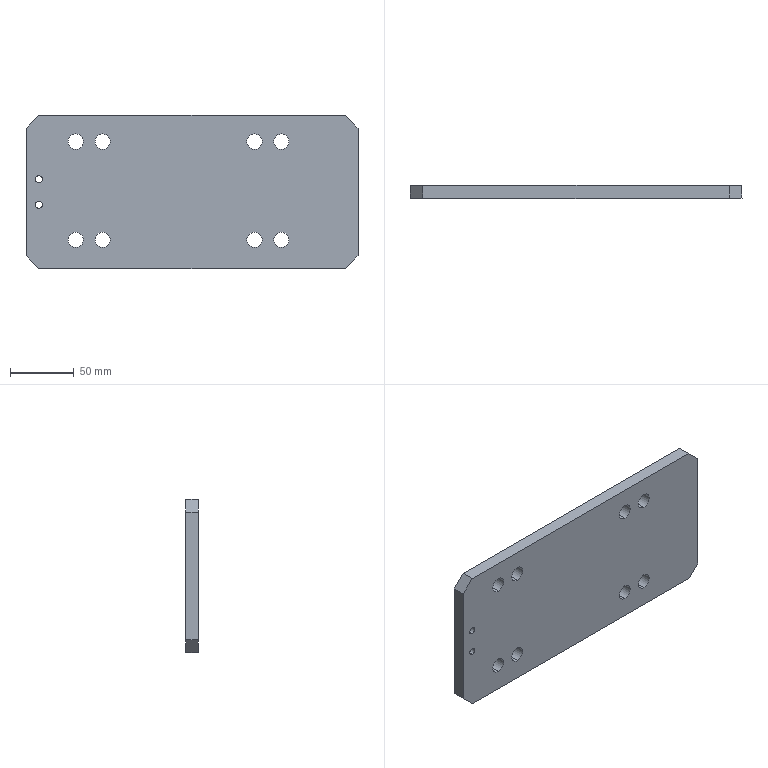Component | SolidWorks | AdsorptionPlate-1 | 1 solid | 30 faces | box 260 x 10.04 x 120 mm | volume 300477 mm3 | cylinder 20 | plane 10 | commonest cylinder face diameters 12 x16 5.5 x4
build123d program:
from build123d import *

# Parameters (mm, degrees)
SKETCH1_W                        = 135
SKETCH1_H                        = 260
BOSS_EXTRUDE1_DEPTH              = 10
M12X1_25_TAPPED_HOLE1_AT_2_COUNT = 2
M12X1_25_TAPPED_HOLE1_AT_2_PITCH = 21
LPATTERN1_COUNT                  = 2
LPATTERN1_PITCH                  = 77
LPATTERN2_COUNT                  = 2
LPATTERN2_PITCH                  = 140
MOVE_FACE1_BY                    = 7.5
MOVE_FACE1_2_BY                  = 7.5
CHAMFER1_SIZE                    = 10
SKETCH4_R                        = 2.75
CUT_EXTRUDE1_DEPTH               = 10


with BuildPart() as part:
    # Sketch1 → Boss-Extrude1 (new body)
    with BuildSketch(Plane.XY):
        Rectangle(SKETCH1_W, SKETCH1_H)
    extrude(amount=BOSS_EXTRUDE1_DEPTH)

    # Sketch2 → M12x1.25 Tapped Hole1 (revolve, cut)
    with BuildSketch(Plane(origin=(37.5, -70, 10), x_dir=(0, -1, 0), z_dir=(1, 0, 0))):
        Polygon((0, 0), (0, 31.355), (6, 27.75), (6, 0), align=None)
    m12x1_25_tapped_hole1 = revolve(axis=Axis((37.5, -70, 16.35), (0, 0, -1)), mode=Mode.SUBTRACT)

    # M12x1.25 Tapped Hole1 at 2: M12x1.25 Tapped Hole1 ×2
    with Locations(*[(0, i * M12X1_25_TAPPED_HOLE1_AT_2_PITCH, 0) for i in range(1, M12X1_25_TAPPED_HOLE1_AT_2_COUNT)]):
        add(m12x1_25_tapped_hole1, mode=Mode.SUBTRACT)

    # LPattern1: M12x1.25 Tapped Hole1 ×2
    with Locations(*[(-i * LPATTERN1_PITCH, 0, 0) for i in range(1, LPATTERN1_COUNT)]):
        add(m12x1_25_tapped_hole1, mode=Mode.SUBTRACT)

    # LPattern1 copy 1 sketch → LPattern1 copy 1 (revolve, cut)
    with BuildSketch(Plane(origin=(-39.5, -49, 10), x_dir=(0, -1, 0), z_dir=(1, 0, 0))):
        Polygon((0, 0), (0, 31.355), (6, 27.75), (6, 0), align=None)
    revolve(axis=Axis((-39.5, -49, 16.35), (0, 0, -1)), mode=Mode.SUBTRACT)

    # LPattern2: M12x1.25 Tapped Hole1 ×2
    with Locations(*[(0, i * LPATTERN2_PITCH, 0) for i in range(1, LPATTERN2_COUNT)]):
        add(m12x1_25_tapped_hole1, mode=Mode.SUBTRACT)

    # LPattern2 copy 1 sketch → LPattern2 copy 1 (revolve, cut)
    with BuildSketch(Plane(origin=(37.5, 91, 10), x_dir=(0, -1, 0), z_dir=(1, 0, 0))):
        Polygon((0, 0), (0, 31.355), (6, 27.75), (6, 0), align=None)
    revolve(axis=Axis((37.5, 91, 16.35), (0, 0, -1)), mode=Mode.SUBTRACT)

    # LPattern2 copy 2 sketch → LPattern2 copy 2 (revolve, cut)
    with BuildSketch(Plane(origin=(-39.5, 70, 10), x_dir=(0, -1, 0), z_dir=(1, 0, 0))):
        Polygon((0, 0), (0, 31.355), (6, 27.75), (6, 0), align=None)
    revolve(axis=Axis((-39.5, 70, 16.35), (0, 0, -1)), mode=Mode.SUBTRACT)

    # LPattern2 copy 3 sketch → LPattern2 copy 3 (revolve, cut)
    with BuildSketch(Plane(origin=(-39.5, 91, 10), x_dir=(0, -1, 0), z_dir=(1, 0, 0))):
        Polygon((0, 0), (0, 31.355), (6, 27.75), (6, 0), align=None)
    revolve(axis=Axis((-39.5, 91, 16.35), (0, 0, -1)), mode=Mode.SUBTRACT)

    # Move Face1: a face moved inward by 7.5
    extrude(part.faces().sort_by_distance((67.5, 0, 5))[0], amount=MOVE_FACE1_BY, dir=(-1, 0, 0), mode=Mode.SUBTRACT)

    # Move Face1 2: a face moved inward by 7.5
    extrude(part.faces().sort_by_distance((-67.5, 0, 5))[0], amount=MOVE_FACE1_2_BY, dir=(1, 0, 0), mode=Mode.SUBTRACT)

    # Chamfer1
    chamfer1_edges = [part.edges().sort_by_distance(p)[0] for p in [
        (-60, 130, 5),
        (60, 130, 5),
        (60, -130, 5),
        (-60, -130, 5),
    ]]
    chamfer(chamfer1_edges, length=CHAMFER1_SIZE)

    # Sketch4 → Cut-Extrude1 (cut)
    with BuildSketch(Plane.XY.offset(10)):
        with Locations((-10, 120)):
            Circle(SKETCH4_R)
        with Locations((10, 120)):
            Circle(SKETCH4_R)
    extrude(amount=-CUT_EXTRUDE1_DEPTH, mode=Mode.SUBTRACT)


solid = part.part

# Placed as in the assembly
solid = solid.moved(Location((1702.164, 3828.72, 1079.241), (-90, -0.008895, 90)))
STEP:
#1=COLOUR_RGB('',0.7922,0.8196,0.9333);
#2=FILL_AREA_STYLE_COLOUR('',#1);
#3=FILL_AREA_STYLE('',(#2));
#4=SURFACE_STYLE_FILL_AREA(#3);
#5=SURFACE_SIDE_STYLE('',(#4));
#6=SURFACE_STYLE_USAGE(.BOTH.,#5);
#7=PRESENTATION_STYLE_ASSIGNMENT((#6));
#8=CARTESIAN_POINT('',(62.29,150.736,41.988));
#9=VERTEX_POINT('',#8);
#10=CARTESIAN_POINT('',(62.29,150.736,42.204));
#11=VERTEX_POINT('',#10);
#12=CARTESIAN_POINT('',(62.29,150.736,42.096));
#13=DIRECTION('',(0.0001552,-1.,0.));
#14=DIRECTION('',(0.,0.,-1.));
#15=AXIS2_PLACEMENT_3D('',#12,#13,#14);
#16=CIRCLE('',#15,0.1083);
#17=EDGE_CURVE('',#9,#11,#16,.T.);
#18=ORIENTED_EDGE('',*,*,#17,.T.);
#19=CARTESIAN_POINT('',(62.29,151.13,42.204));
#20=VERTEX_POINT('',#19);
#21=CARTESIAN_POINT('',(62.29,150.43,42.204));
#22=DIRECTION('',(-0.0001552,1.,-0.));
#23=VECTOR('',#22,39.37);
#24=LINE('',#21,#23);
#25=EDGE_CURVE('',#11,#20,#24,.T.);
#26=ORIENTED_EDGE('',*,*,#25,.T.);
#27=CARTESIAN_POINT('',(62.29,151.13,41.988));
#28=VERTEX_POINT('',#27);
#29=CARTESIAN_POINT('',(62.29,151.13,42.096));
#30=DIRECTION('',(-0.0001552,1.,-0.));
#31=DIRECTION('',(0.,0.,-1.));
#32=AXIS2_PLACEMENT_3D('',#29,#30,#31);
#33=CIRCLE('',#32,0.1083);
#34=EDGE_CURVE('',#20,#28,#33,.T.);
#35=ORIENTED_EDGE('',*,*,#34,.T.);
#36=CARTESIAN_POINT('',(62.29,150.43,41.988));
#37=DIRECTION('',(-0.0001552,1.,-0.));
#38=VECTOR('',#37,39.37);
#39=LINE('',#36,#38);
#40=EDGE_CURVE('',#9,#28,#39,.T.);
#41=ORIENTED_EDGE('',*,*,#40,.F.);
#42=EDGE_LOOP('',(#18,#26,#35,#41));
#43=FACE_OUTER_BOUND('',#42,.T.);
#44=CARTESIAN_POINT('',(62.29,150.43,42.096));
#45=DIRECTION('',(-0.0001552,1.,-0.));
#46=DIRECTION('',(0.,0.,-1.));
#47=AXIS2_PLACEMENT_3D('',#44,#45,#46);
#48=CYLINDRICAL_SURFACE('',#47,0.1083);
#49=ADVANCED_FACE('',(#43),#48,.F.);
#50=CARTESIAN_POINT('',(62.29,150.736,42.775));
#51=VERTEX_POINT('',#50);
#52=CARTESIAN_POINT('',(62.29,150.736,42.992));
#53=VERTEX_POINT('',#52);
#54=CARTESIAN_POINT('',(62.29,150.736,42.884));
#55=DIRECTION('',(0.0001552,-1.,0.));
#56=DIRECTION('',(0.,0.,-1.));
#57=AXIS2_PLACEMENT_3D('',#54,#55,#56);
#58=CIRCLE('',#57,0.1083);
#59=EDGE_CURVE('',#51,#53,#58,.T.);
#60=ORIENTED_EDGE('',*,*,#59,.T.);
#61=CARTESIAN_POINT('',(62.29,151.13,42.992));
#62=VERTEX_POINT('',#61);
#63=CARTESIAN_POINT('',(62.29,150.43,42.992));
#64=DIRECTION('',(-0.0001552,1.,-0.));
#65=VECTOR('',#64,39.37);
#66=LINE('',#63,#65);
#67=EDGE_CURVE('',#53,#62,#66,.T.);
#68=ORIENTED_EDGE('',*,*,#67,.T.);
#69=CARTESIAN_POINT('',(62.29,151.13,42.775));
#70=VERTEX_POINT('',#69);
#71=CARTESIAN_POINT('',(62.29,151.13,42.884));
#72=DIRECTION('',(-0.0001552,1.,-0.));
#73=DIRECTION('',(0.,0.,-1.));
#74=AXIS2_PLACEMENT_3D('',#71,#72,#73);
#75=CIRCLE('',#74,0.1083);
#76=EDGE_CURVE('',#62,#70,#75,.T.);
#77=ORIENTED_EDGE('',*,*,#76,.T.);
#78=CARTESIAN_POINT('',(62.29,150.43,42.775));
#79=DIRECTION('',(-0.0001552,1.,-0.));
#80=VECTOR('',#79,39.37);
#81=LINE('',#78,#80);
#82=EDGE_CURVE('',#51,#70,#81,.T.);
#83=ORIENTED_EDGE('',*,*,#82,.F.);
#84=EDGE_LOOP('',(#60,#68,#77,#83));
#85=FACE_OUTER_BOUND('',#84,.T.);
#86=CARTESIAN_POINT('',(62.29,150.43,42.884));
#87=DIRECTION('',(-0.0001552,1.,-0.));
#88=DIRECTION('',(0.,0.,-1.));
#89=AXIS2_PLACEMENT_3D('',#86,#87,#88);
#90=CYLINDRICAL_SURFACE('',#89,0.1083);
#91=ADVANCED_FACE('',(#85),#90,.F.);
#92=CARTESIAN_POINT('',(64.258,150.737,44.281));
#93=VERTEX_POINT('',#92);
#94=CARTESIAN_POINT('',(64.258,150.737,43.809));
#95=VERTEX_POINT('',#94);
#96=CARTESIAN_POINT('',(64.258,150.737,44.045));
#97=DIRECTION('',(-0.0001552,1.,-0.));
#98=DIRECTION('',(0.,0.,-1.));
#99=AXIS2_PLACEMENT_3D('',#96,#97,#98);
#100=CIRCLE('',#99,0.2362);
#101=EDGE_CURVE('',#93,#95,#100,.T.);
#102=ORIENTED_EDGE('',*,*,#101,.F.);
#103=CARTESIAN_POINT('',(64.258,151.13,44.281));
#104=VERTEX_POINT('',#103);
#105=CARTESIAN_POINT('',(64.258,151.13,44.281));
#106=DIRECTION('',(-0.0001552,1.,-0.));
#107=VECTOR('',#106,39.37);
#108=LINE('',#105,#107);
#109=EDGE_CURVE('',#93,#104,#108,.T.);
#110=ORIENTED_EDGE('',*,*,#109,.T.);
#111=CARTESIAN_POINT('',(64.258,151.13,43.809));
#112=VERTEX_POINT('',#111);
#113=CARTESIAN_POINT('',(64.258,151.13,44.045));
#114=DIRECTION('',(-0.0001552,1.,-0.));
#115=DIRECTION('',(0.,0.,-1.));
#116=AXIS2_PLACEMENT_3D('',#113,#114,#115);
#117=CIRCLE('',#116,0.2362);
#118=EDGE_CURVE('',#104,#112,#117,.T.);
#119=ORIENTED_EDGE('',*,*,#118,.T.);
#120=CARTESIAN_POINT('',(64.258,151.13,43.809));
#121=DIRECTION('',(-0.0001552,1.,-0.));
#122=VECTOR('',#121,39.37);
#123=LINE('',#120,#122);
#124=EDGE_CURVE('',#95,#112,#123,.T.);
#125=ORIENTED_EDGE('',*,*,#124,.F.);
#126=EDGE_LOOP('',(#102,#110,#119,#125));
#127=FACE_OUTER_BOUND('',#126,.T.);
#128=CARTESIAN_POINT('',(64.258,151.13,44.045));
#129=DIRECTION('',(-0.0001552,1.,-0.));
#130=DIRECTION('',(0.,0.,-1.));
#131=AXIS2_PLACEMENT_3D('',#128,#129,#130);
#132=CYLINDRICAL_SURFACE('',#131,0.2362);
#133=ADVANCED_FACE('',(#127),#132,.F.);
#134=CARTESIAN_POINT('',(64.258,150.737,41.25));
#135=VERTEX_POINT('',#134);
#136=CARTESIAN_POINT('',(64.258,150.737,40.777));
#137=VERTEX_POINT('',#136);
#138=CARTESIAN_POINT('',(64.258,150.737,41.013));
#139=DIRECTION('',(-0.0001552,1.,-0.));
#140=DIRECTION('',(0.,0.,-1.));
#141=AXIS2_PLACEMENT_3D('',#138,#139,#140);
#142=CIRCLE('',#141,0.2362);
#143=EDGE_CURVE('',#135,#137,#142,.T.);
#144=ORIENTED_EDGE('',*,*,#143,.F.);
#145=CARTESIAN_POINT('',(64.258,151.13,41.25));
#146=VERTEX_POINT('',#145);
#147=CARTESIAN_POINT('',(64.258,151.13,41.25));
#148=DIRECTION('',(-0.0001552,1.,-0.));
#149=VECTOR('',#148,39.37);
#150=LINE('',#147,#149);
#151=EDGE_CURVE('',#135,#146,#150,.T.);
#152=ORIENTED_EDGE('',*,*,#151,.T.);
#153=CARTESIAN_POINT('',(64.258,151.13,40.777));
#154=VERTEX_POINT('',#153);
#155=CARTESIAN_POINT('',(64.258,151.13,41.013));
#156=DIRECTION('',(-0.0001552,1.,-0.));
#157=DIRECTION('',(0.,0.,-1.));
#158=AXIS2_PLACEMENT_3D('',#155,#156,#157);
#159=CIRCLE('',#158,0.2362);
#160=EDGE_CURVE('',#146,#154,#159,.T.);
#161=ORIENTED_EDGE('',*,*,#160,.T.);
#162=CARTESIAN_POINT('',(64.258,151.13,40.777));
#163=DIRECTION('',(-0.0001552,1.,-0.));
#164=VECTOR('',#163,39.37);
#165=LINE('',#162,#164);
#166=EDGE_CURVE('',#137,#154,#165,.T.);
#167=ORIENTED_EDGE('',*,*,#166,.F.);
#168=EDGE_LOOP('',(#144,#152,#161,#167));
#169=FACE_OUTER_BOUND('',#168,.T.);
#170=CARTESIAN_POINT('',(64.258,151.13,41.013));
#171=DIRECTION('',(-0.0001552,1.,-0.));
#172=DIRECTION('',(0.,0.,-1.));
#173=AXIS2_PLACEMENT_3D('',#170,#171,#172);
#174=CYLINDRICAL_SURFACE('',#173,0.2362);
#175=ADVANCED_FACE('',(#169),#174,.F.);
#176=CARTESIAN_POINT('',(63.432,150.736,41.25));
#177=VERTEX_POINT('',#176);
#178=CARTESIAN_POINT('',(63.432,150.736,40.777));
#179=VERTEX_POINT('',#178);
#180=CARTESIAN_POINT('',(63.432,150.736,41.013));
#181=DIRECTION('',(-0.0001552,1.,-0.));
#182=DIRECTION('',(0.,0.,-1.));
#183=AXIS2_PLACEMENT_3D('',#180,#181,#182);
#184=CIRCLE('',#183,0.2362);
#185=EDGE_CURVE('',#177,#179,#184,.T.);
#186=ORIENTED_EDGE('',*,*,#185,.F.);
#187=CARTESIAN_POINT('',(63.432,151.13,41.25));
#188=VERTEX_POINT('',#187);
#189=CARTESIAN_POINT('',(63.432,151.13,41.25));
#190=DIRECTION('',(-0.0001552,1.,-0.));
#191=VECTOR('',#190,39.37);
#192=LINE('',#189,#191);
#193=EDGE_CURVE('',#177,#188,#192,.T.);
#194=ORIENTED_EDGE('',*,*,#193,.T.);
#195=CARTESIAN_POINT('',(63.432,151.13,40.777));
#196=VERTEX_POINT('',#195);
#197=CARTESIAN_POINT('',(63.432,151.13,41.013));
#198=DIRECTION('',(-0.0001552,1.,-0.));
#199=DIRECTION('',(0.,0.,-1.));
#200=AXIS2_PLACEMENT_3D('',#197,#198,#199);
#201=CIRCLE('',#200,0.2362);
#202=EDGE_CURVE('',#188,#196,#201,.T.);
#203=ORIENTED_EDGE('',*,*,#202,.T.);
#204=CARTESIAN_POINT('',(63.432,151.13,40.777));
#205=DIRECTION('',(-0.0001552,1.,-0.));
#206=VECTOR('',#205,39.37);
#207=LINE('',#204,#206);
#208=EDGE_CURVE('',#179,#196,#207,.T.);
#209=ORIENTED_EDGE('',*,*,#208,.F.);
#210=EDGE_LOOP('',(#186,#194,#203,#209));
#211=FACE_OUTER_BOUND('',#210,.T.);
#212=CARTESIAN_POINT('',(63.432,151.13,41.013));
#213=DIRECTION('',(-0.0001552,1.,-0.));
#214=DIRECTION('',(0.,0.,-1.));
#215=AXIS2_PLACEMENT_3D('',#212,#213,#214);
#216=CYLINDRICAL_SURFACE('',#215,0.2362);
#217=ADVANCED_FACE('',(#211),#216,.F.);
#218=CARTESIAN_POINT('',(63.432,150.736,44.281));
#219=VERTEX_POINT('',#218);
#220=CARTESIAN_POINT('',(63.432,150.736,43.809));
#221=VERTEX_POINT('',#220);
#222=CARTESIAN_POINT('',(63.432,150.736,44.045));
#223=DIRECTION('',(-0.0001552,1.,-0.));
#224=DIRECTION('',(0.,0.,-1.));
#225=AXIS2_PLACEMENT_3D('',#222,#223,#224);
#226=CIRCLE('',#225,0.2362);
#227=EDGE_CURVE('',#219,#221,#226,.T.);
#228=ORIENTED_EDGE('',*,*,#227,.F.);
#229=CARTESIAN_POINT('',(63.432,151.13,44.281));
#230=VERTEX_POINT('',#229);
#231=CARTESIAN_POINT('',(63.432,151.13,44.281));
#232=DIRECTION('',(-0.0001552,1.,-0.));
#233=VECTOR('',#232,39.37);
#234=LINE('',#231,#233);
#235=EDGE_CURVE('',#219,#230,#234,.T.);
#236=ORIENTED_EDGE('',*,*,#235,.T.);
#237=CARTESIAN_POINT('',(63.432,151.13,43.809));
#238=VERTEX_POINT('',#237);
#239=CARTESIAN_POINT('',(63.432,151.13,44.045));
#240=DIRECTION('',(-0.0001552,1.,-0.));
#241=DIRECTION('',(0.,0.,-1.));
#242=AXIS2_PLACEMENT_3D('',#239,#240,#241);
#243=CIRCLE('',#242,0.2362);
#244=EDGE_CURVE('',#230,#238,#243,.T.);
#245=ORIENTED_EDGE('',*,*,#244,.T.);
#246=CARTESIAN_POINT('',(63.432,151.13,43.809));
#247=DIRECTION('',(-0.0001552,1.,-0.));
#248=VECTOR('',#247,39.37);
#249=LINE('',#246,#248);
#250=EDGE_CURVE('',#221,#238,#249,.T.);
#251=ORIENTED_EDGE('',*,*,#250,.F.);
#252=EDGE_LOOP('',(#228,#236,#245,#251));
#253=FACE_OUTER_BOUND('',#252,.T.);
#254=CARTESIAN_POINT('',(63.432,151.13,44.045));
#255=DIRECTION('',(-0.0001552,1.,-0.));
#256=DIRECTION('',(0.,0.,-1.));
#257=AXIS2_PLACEMENT_3D('',#254,#255,#256);
#258=CYLINDRICAL_SURFACE('',#257,0.2362);
#259=ADVANCED_FACE('',(#253),#258,.F.);
#260=CARTESIAN_POINT('',(68.943,150.737,44.281));
#261=VERTEX_POINT('',#260);
#262=CARTESIAN_POINT('',(68.943,150.737,43.809));
#263=VERTEX_POINT('',#262);
#264=CARTESIAN_POINT('',(68.943,150.737,44.045));
#265=DIRECTION('',(-0.0001552,1.,-0.));
#266=DIRECTION('',(0.,0.,-1.));
#267=AXIS2_PLACEMENT_3D('',#264,#265,#266);
#268=CIRCLE('',#267,0.2362);
#269=EDGE_CURVE('',#261,#263,#268,.T.);
#270=ORIENTED_EDGE('',*,*,#269,.F.);
#271=CARTESIAN_POINT('',(68.943,151.131,44.281));
#272=VERTEX_POINT('',#271);
#273=CARTESIAN_POINT('',(68.943,151.131,44.281));
#274=DIRECTION('',(-0.0001552,1.,-0.));
#275=VECTOR('',#274,39.37);
#276=LINE('',#273,#275);
#277=EDGE_CURVE('',#261,#272,#276,.T.);
#278=ORIENTED_EDGE('',*,*,#277,.T.);
#279=CARTESIAN_POINT('',(68.943,151.131,43.809));
#280=VERTEX_POINT('',#279);
#281=CARTESIAN_POINT('',(68.943,151.131,44.045));
#282=DIRECTION('',(-0.0001552,1.,-0.));
#283=DIRECTION('',(0.,0.,-1.));
#284=AXIS2_PLACEMENT_3D('',#281,#282,#283);
#285=CIRCLE('',#284,0.2362);
#286=EDGE_CURVE('',#272,#280,#285,.T.);
#287=ORIENTED_EDGE('',*,*,#286,.T.);
#288=CARTESIAN_POINT('',(68.943,151.131,43.809));
#289=DIRECTION('',(-0.0001552,1.,-0.));
#290=VECTOR('',#289,39.37);
#291=LINE('',#288,#290);
#292=EDGE_CURVE('',#263,#280,#291,.T.);
#293=ORIENTED_EDGE('',*,*,#292,.F.);
#294=EDGE_LOOP('',(#270,#278,#287,#293));
#295=FACE_OUTER_BOUND('',#294,.T.);
#296=CARTESIAN_POINT('',(68.943,151.131,44.045));
#297=DIRECTION('',(-0.0001552,1.,-0.));
#298=DIRECTION('',(0.,0.,-1.));
#299=AXIS2_PLACEMENT_3D('',#296,#297,#298);
#300=CYLINDRICAL_SURFACE('',#299,0.2362);
#301=ADVANCED_FACE('',(#295),#300,.F.);
#302=CARTESIAN_POINT('',(69.77,150.737,44.281));
#303=VERTEX_POINT('',#302);
#304=CARTESIAN_POINT('',(69.77,150.737,43.809));
#305=VERTEX_POINT('',#304);
#306=CARTESIAN_POINT('',(69.77,150.737,44.045));
#307=DIRECTION('',(-0.0001552,1.,-0.));
#308=DIRECTION('',(0.,0.,-1.));
#309=AXIS2_PLACEMENT_3D('',#306,#307,#308);
#310=CIRCLE('',#309,0.2362);
#311=EDGE_CURVE('',#303,#305,#310,.T.);
#312=ORIENTED_EDGE('',*,*,#311,.F.);
#313=CARTESIAN_POINT('',(69.77,151.131,44.281));
#314=VERTEX_POINT('',#313);
#315=CARTESIAN_POINT('',(69.77,151.131,44.281));
#316=DIRECTION('',(-0.0001552,1.,-0.));
#317=VECTOR('',#316,39.37);
#318=LINE('',#315,#317);
#319=EDGE_CURVE('',#303,#314,#318,.T.);
#320=ORIENTED_EDGE('',*,*,#319,.T.);
#321=CARTESIAN_POINT('',(69.77,151.131,43.809));
#322=VERTEX_POINT('',#321);
#323=CARTESIAN_POINT('',(69.77,151.131,44.045));
#324=DIRECTION('',(-0.0001552,1.,-0.));
#325=DIRECTION('',(0.,0.,-1.));
#326=AXIS2_PLACEMENT_3D('',#323,#324,#325);
#327=CIRCLE('',#326,0.2362);
#328=EDGE_CURVE('',#314,#322,#327,.T.);
#329=ORIENTED_EDGE('',*,*,#328,.T.);
#330=CARTESIAN_POINT('',(69.77,151.131,43.809));
#331=DIRECTION('',(-0.0001552,1.,-0.));
#332=VECTOR('',#331,39.37);
#333=LINE('',#330,#332);
#334=EDGE_CURVE('',#305,#322,#333,.T.);
#335=ORIENTED_EDGE('',*,*,#334,.F.);
#336=EDGE_LOOP('',(#312,#320,#329,#335));
#337=FACE_OUTER_BOUND('',#336,.T.);
#338=CARTESIAN_POINT('',(69.77,151.131,44.045));
#339=DIRECTION('',(-0.0001552,1.,-0.));
#340=DIRECTION('',(0.,0.,-1.));
#341=AXIS2_PLACEMENT_3D('',#338,#339,#340);
#342=CYLINDRICAL_SURFACE('',#341,0.2362);
#343=ADVANCED_FACE('',(#337),#342,.F.);
#344=CARTESIAN_POINT('',(69.77,150.737,41.25));
#345=VERTEX_POINT('',#344);
#346=CARTESIAN_POINT('',(69.77,150.737,40.777));
#347=VERTEX_POINT('',#346);
#348=CARTESIAN_POINT('',(69.77,150.737,41.013));
#349=DIRECTION('',(-0.0001552,1.,-0.));
#350=DIRECTION('',(0.,0.,-1.));
#351=AXIS2_PLACEMENT_3D('',#348,#349,#350);
#352=CIRCLE('',#351,0.2362);
#353=EDGE_CURVE('',#345,#347,#352,.T.);
#354=ORIENTED_EDGE('',*,*,#353,.F.);
#355=CARTESIAN_POINT('',(69.77,151.131,41.25));
#356=VERTEX_POINT('',#355);
#357=CARTESIAN_POINT('',(69.77,151.131,41.25));
#358=DIRECTION('',(-0.0001552,1.,-0.));
#359=VECTOR('',#358,39.37);
#360=LINE('',#357,#359);
#361=EDGE_CURVE('',#345,#356,#360,.T.);
#362=ORIENTED_EDGE('',*,*,#361,.T.);
#363=CARTESIAN_POINT('',(69.77,151.131,40.777));
#364=VERTEX_POINT('',#363);
#365=CARTESIAN_POINT('',(69.77,151.131,41.013));
#366=DIRECTION('',(-0.0001552,1.,-0.));
#367=DIRECTION('',(0.,0.,-1.));
#368=AXIS2_PLACEMENT_3D('',#365,#366,#367);
#369=CIRCLE('',#368,0.2362);
#370=EDGE_CURVE('',#356,#364,#369,.T.);
#371=ORIENTED_EDGE('',*,*,#370,.T.);
#372=CARTESIAN_POINT('',(69.77,151.131,40.777));
#373=DIRECTION('',(-0.0001552,1.,-0.));
#374=VECTOR('',#373,39.37);
#375=LINE('',#372,#374);
#376=EDGE_CURVE('',#347,#364,#375,.T.);
#377=ORIENTED_EDGE('',*,*,#376,.F.);
#378=EDGE_LOOP('',(#354,#362,#371,#377));
#379=FACE_OUTER_BOUND('',#378,.T.);
#380=CARTESIAN_POINT('',(69.77,151.131,41.013));
#381=DIRECTION('',(-0.0001552,1.,-0.));
#382=DIRECTION('',(0.,0.,-1.));
#383=AXIS2_PLACEMENT_3D('',#380,#381,#382);
#384=CYLINDRICAL_SURFACE('',#383,0.2362);
#385=ADVANCED_FACE('',(#379),#384,.F.);
#386=CARTESIAN_POINT('',(68.943,150.737,41.25));
#387=VERTEX_POINT('',#386);
#388=CARTESIAN_POINT('',(68.943,150.737,40.777));
#389=VERTEX_POINT('',#388);
#390=CARTESIAN_POINT('',(68.943,150.737,41.013));
#391=DIRECTION('',(-0.0001552,1.,-0.));
#392=DIRECTION('',(0.,0.,-1.));
#393=AXIS2_PLACEMENT_3D('',#390,#391,#392);
#394=CIRCLE('',#393,0.2362);
#395=EDGE_CURVE('',#387,#389,#394,.T.);
#396=ORIENTED_EDGE('',*,*,#395,.F.);
#397=CARTESIAN_POINT('',(68.943,151.131,41.25));
#398=VERTEX_POINT('',#397);
#399=CARTESIAN_POINT('',(68.943,151.131,41.25));
#400=DIRECTION('',(-0.0001552,1.,-0.));
#401=VECTOR('',#400,39.37);
#402=LINE('',#399,#401);
#403=EDGE_CURVE('',#387,#398,#402,.T.);
#404=ORIENTED_EDGE('',*,*,#403,.T.);
#405=CARTESIAN_POINT('',(68.943,151.131,40.777));
#406=VERTEX_POINT('',#405);
#407=CARTESIAN_POINT('',(68.943,151.131,41.013));
#408=DIRECTION('',(-0.0001552,1.,-0.));
#409=DIRECTION('',(0.,0.,-1.));
#410=AXIS2_PLACEMENT_3D('',#407,#408,#409);
#411=CIRCLE('',#410,0.2362);
#412=EDGE_CURVE('',#398,#406,#411,.T.);
#413=ORIENTED_EDGE('',*,*,#412,.T.);
#414=CARTESIAN_POINT('',(68.943,151.131,40.777));
#415=DIRECTION('',(-0.0001552,1.,-0.));
#416=VECTOR('',#415,39.37);
#417=LINE('',#414,#416);
#418=EDGE_CURVE('',#389,#406,#417,.T.);
#419=ORIENTED_EDGE('',*,*,#418,.F.);
#420=EDGE_LOOP('',(#396,#404,#413,#419));
#421=FACE_OUTER_BOUND('',#420,.T.);
#422=CARTESIAN_POINT('',(68.943,151.131,41.013));
#423=DIRECTION('',(-0.0001552,1.,-0.));
#424=DIRECTION('',(0.,0.,-1.));
#425=AXIS2_PLACEMENT_3D('',#422,#423,#424);
#426=CYLINDRICAL_SURFACE('',#425,0.2362);
#427=ADVANCED_FACE('',(#421),#426,.F.);
#428=CARTESIAN_POINT('',(62.29,151.13,44.852));
#429=VERTEX_POINT('',#428);
#430=CARTESIAN_POINT('',(71.739,151.131,44.852));
#431=VERTEX_POINT('',#430);
#432=CARTESIAN_POINT('',(72.132,151.132,44.852));
#433=DIRECTION('',(1.,0.0001552,0.));
#434=VECTOR('',#433,39.37);
#435=LINE('',#432,#434);
#436=EDGE_CURVE('',#429,#431,#435,.T.);
#437=ORIENTED_EDGE('',*,*,#436,.F.);
#438=CARTESIAN_POINT('',(62.29,150.736,44.852));
#439=VERTEX_POINT('',#438);
#440=CARTESIAN_POINT('',(62.29,151.13,44.852));
#441=DIRECTION('',(0.0001552,-1.,0.));
#442=VECTOR('',#441,39.37);
#443=LINE('',#440,#442);
#444=EDGE_CURVE('',#429,#439,#443,.T.);
#445=ORIENTED_EDGE('',*,*,#444,.T.);
#446=CARTESIAN_POINT('',(71.739,150.738,44.852));
#447=VERTEX_POINT('',#446);
#448=CARTESIAN_POINT('',(72.132,150.738,44.852));
#449=DIRECTION('',(1.,0.0001552,0.));
#450=VECTOR('',#449,39.37);
#451=LINE('',#448,#450);
#452=EDGE_CURVE('',#439,#447,#451,.T.);
#453=ORIENTED_EDGE('',*,*,#452,.T.);
#454=CARTESIAN_POINT('',(71.739,151.131,44.852));
#455=DIRECTION('',(-0.0001552,1.,-0.));
#456=VECTOR('',#455,39.37);
#457=LINE('',#454,#456);
#458=EDGE_CURVE('',#447,#431,#457,.T.);
#459=ORIENTED_EDGE('',*,*,#458,.T.);
#460=EDGE_LOOP('',(#437,#445,#453,#459));
#461=FACE_OUTER_BOUND('',#460,.T.);
#462=CARTESIAN_POINT('',(72.132,151.132,44.852));
#463=DIRECTION('',(0.,-0.,-1.));
#464=DIRECTION('',(0.0001552,-1.,0.));
#465=AXIS2_PLACEMENT_3D('',#462,#463,#464);
#466=PLANE('',#465);
#467=ADVANCED_FACE('',(#461),#466,.F.);
#468=CARTESIAN_POINT('',(72.132,150.738,44.458));
#469=VERTEX_POINT('',#468);
#470=CARTESIAN_POINT('',(72.132,150.738,40.521));
#471=VERTEX_POINT('',#470);
#472=CARTESIAN_POINT('',(72.132,150.738,39.832));
#473=DIRECTION('',(0.,-0.,-1.));
#474=VECTOR('',#473,39.37);
#475=LINE('',#472,#474);
#476=EDGE_CURVE('',#469,#471,#475,.T.);
#477=ORIENTED_EDGE('',*,*,#476,.T.);
#478=CARTESIAN_POINT('',(72.132,151.132,40.521));
#479=VERTEX_POINT('',#478);
#480=CARTESIAN_POINT('',(72.132,151.132,40.521));
#481=DIRECTION('',(-0.0001552,1.,-0.));
#482=VECTOR('',#481,39.37);
#483=LINE('',#480,#482);
#484=EDGE_CURVE('',#471,#479,#483,.T.);
#485=ORIENTED_EDGE('',*,*,#484,.T.);
#486=CARTESIAN_POINT('',(72.132,151.132,44.458));
#487=VERTEX_POINT('',#486);
#488=CARTESIAN_POINT('',(72.132,151.132,39.832));
#489=DIRECTION('',(0.,-0.,-1.));
#490=VECTOR('',#489,39.37);
#491=LINE('',#488,#490);
#492=EDGE_CURVE('',#487,#479,#491,.T.);
#493=ORIENTED_EDGE('',*,*,#492,.F.);
#494=CARTESIAN_POINT('',(72.132,151.132,44.458));
#495=DIRECTION('',(0.0001552,-1.,0.));
#496=VECTOR('',#495,39.37);
#497=LINE('',#494,#496);
#498=EDGE_CURVE('',#487,#469,#497,.T.);
#499=ORIENTED_EDGE('',*,*,#498,.T.);
#500=EDGE_LOOP('',(#477,#485,#493,#499));
#501=FACE_OUTER_BOUND('',#500,.T.);
#502=CARTESIAN_POINT('',(72.132,151.132,39.832));
#503=DIRECTION('',(-1.,-0.0001552,-0.));
#504=DIRECTION('',(-0.0001552,1.,-0.));
#505=AXIS2_PLACEMENT_3D('',#502,#503,#504);
#506=PLANE('',#505);
#507=ADVANCED_FACE('',(#501),#506,.F.);
#508=CARTESIAN_POINT('',(71.739,150.738,40.128));
#509=VERTEX_POINT('',#508);
#510=CARTESIAN_POINT('',(62.29,150.736,40.128));
#511=VERTEX_POINT('',#510);
#512=CARTESIAN_POINT('',(72.132,150.738,40.128));
#513=DIRECTION('',(-1.,-0.0001552,-0.));
#514=VECTOR('',#513,39.37);
#515=LINE('',#512,#514);
#516=EDGE_CURVE('',#509,#511,#515,.T.);
#517=ORIENTED_EDGE('',*,*,#516,.T.);
#518=CARTESIAN_POINT('',(62.29,151.13,40.128));
#519=VERTEX_POINT('',#518);
#520=CARTESIAN_POINT('',(62.29,151.13,40.128));
#521=DIRECTION('',(-0.0001552,1.,-0.));
#522=VECTOR('',#521,39.37);
#523=LINE('',#520,#522);
#524=EDGE_CURVE('',#511,#519,#523,.T.);
#525=ORIENTED_EDGE('',*,*,#524,.T.);
#526=CARTESIAN_POINT('',(71.739,151.131,40.128));
#527=VERTEX_POINT('',#526);
#528=CARTESIAN_POINT('',(72.132,151.132,40.128));
#529=DIRECTION('',(-1.,-0.0001552,-0.));
#530=VECTOR('',#529,39.37);
#531=LINE('',#528,#530);
#532=EDGE_CURVE('',#527,#519,#531,.T.);
#533=ORIENTED_EDGE('',*,*,#532,.F.);
#534=CARTESIAN_POINT('',(71.739,151.131,40.128));
#535=DIRECTION('',(0.0001552,-1.,0.));
#536=VECTOR('',#535,39.37);
#537=LINE('',#534,#536);
#538=EDGE_CURVE('',#527,#509,#537,.T.);
#539=ORIENTED_EDGE('',*,*,#538,.T.);
#540=EDGE_LOOP('',(#517,#525,#533,#539));
#541=FACE_OUTER_BOUND('',#540,.T.);
#542=CARTESIAN_POINT('',(72.132,151.132,40.128));
#543=DIRECTION('',(-0.,0.,1.));
#544=DIRECTION('',(-0.0001552,1.,-0.));
#545=AXIS2_PLACEMENT_3D('',#542,#543,#544);
#546=PLANE('',#545);
#547=ADVANCED_FACE('',(#541),#546,.F.);
#548=CARTESIAN_POINT('',(61.896,150.736,40.521));
#549=VERTEX_POINT('',#548);
#550=CARTESIAN_POINT('',(61.896,150.736,44.458));
#551=VERTEX_POINT('',#550);
#552=CARTESIAN_POINT('',(61.896,150.736,39.832));
#553=DIRECTION('',(0.,0.,1.));
#554=VECTOR('',#553,39.37);
#555=LINE('',#552,#554);
#556=EDGE_CURVE('',#549,#551,#555,.T.);
#557=ORIENTED_EDGE('',*,*,#556,.T.);
#558=CARTESIAN_POINT('',(61.896,151.13,44.458));
#559=VERTEX_POINT('',#558);
#560=CARTESIAN_POINT('',(61.896,151.13,44.458));
#561=DIRECTION('',(-0.0001552,1.,-0.));
#562=VECTOR('',#561,39.37);
#563=LINE('',#560,#562);
#564=EDGE_CURVE('',#551,#559,#563,.T.);
#565=ORIENTED_EDGE('',*,*,#564,.T.);
#566=CARTESIAN_POINT('',(61.896,151.13,40.521));
#567=VERTEX_POINT('',#566);
#568=CARTESIAN_POINT('',(61.896,151.13,39.832));
#569=DIRECTION('',(0.,0.,1.));
#570=VECTOR('',#569,39.37);
#571=LINE('',#568,#570);
#572=EDGE_CURVE('',#567,#559,#571,.T.);
#573=ORIENTED_EDGE('',*,*,#572,.F.);
#574=CARTESIAN_POINT('',(61.896,151.13,40.521));
#575=DIRECTION('',(0.0001552,-1.,0.));
#576=VECTOR('',#575,39.37);
#577=LINE('',#574,#576);
#578=EDGE_CURVE('',#567,#549,#577,.T.);
#579=ORIENTED_EDGE('',*,*,#578,.T.);
#580=EDGE_LOOP('',(#557,#565,#573,#579));
#581=FACE_OUTER_BOUND('',#580,.T.);
#582=CARTESIAN_POINT('',(61.896,151.13,39.832));
#583=DIRECTION('',(1.,0.0001552,-0.));
#584=DIRECTION('',(-0.,-0.,-1.));
#585=AXIS2_PLACEMENT_3D('',#582,#583,#584);
#586=PLANE('',#585);
#587=ADVANCED_FACE('',(#581),#586,.F.);
#588=CARTESIAN_POINT('',(62.29,151.13,42.096));
#589=DIRECTION('',(-0.0001552,1.,-0.));
#590=DIRECTION('',(0.,0.,-1.));
#591=AXIS2_PLACEMENT_3D('',#588,#589,#590);
#592=CIRCLE('',#591,0.1083);
#593=EDGE_CURVE('',#28,#20,#592,.T.);
#594=ORIENTED_EDGE('',*,*,#593,.F.);
#595=ORIENTED_EDGE('',*,*,#34,.F.);
#596=EDGE_LOOP('',(#594,#595));
#597=FACE_BOUND('',#596,.T.);
#598=CARTESIAN_POINT('',(62.29,151.13,42.884));
#599=DIRECTION('',(-0.0001552,1.,-0.));
#600=DIRECTION('',(0.,0.,-1.));
#601=AXIS2_PLACEMENT_3D('',#598,#599,#600);
#602=CIRCLE('',#601,0.1083);
#603=EDGE_CURVE('',#70,#62,#602,.T.);
#604=ORIENTED_EDGE('',*,*,#603,.F.);
#605=ORIENTED_EDGE('',*,*,#76,.F.);
#606=EDGE_LOOP('',(#604,#605));
#607=FACE_BOUND('',#606,.T.);
#608=CARTESIAN_POINT('',(64.258,151.13,44.045));
#609=DIRECTION('',(-0.0001552,1.,-0.));
#610=DIRECTION('',(0.,0.,-1.));
#611=AXIS2_PLACEMENT_3D('',#608,#609,#610);
#612=CIRCLE('',#611,0.2362);
#613=EDGE_CURVE('',#112,#104,#612,.T.);
#614=ORIENTED_EDGE('',*,*,#613,.F.);
#615=ORIENTED_EDGE('',*,*,#118,.F.);
#616=EDGE_LOOP('',(#614,#615));
#617=FACE_BOUND('',#616,.T.);
#618=CARTESIAN_POINT('',(64.258,151.13,41.013));
#619=DIRECTION('',(-0.0001552,1.,-0.));
#620=DIRECTION('',(0.,0.,-1.));
#621=AXIS2_PLACEMENT_3D('',#618,#619,#620);
#622=CIRCLE('',#621,0.2362);
#623=EDGE_CURVE('',#154,#146,#622,.T.);
#624=ORIENTED_EDGE('',*,*,#623,.F.);
#625=ORIENTED_EDGE('',*,*,#160,.F.);
#626=EDGE_LOOP('',(#624,#625));
#627=FACE_BOUND('',#626,.T.);
#628=CARTESIAN_POINT('',(63.432,151.13,41.013));
#629=DIRECTION('',(-0.0001552,1.,-0.));
#630=DIRECTION('',(0.,0.,-1.));
#631=AXIS2_PLACEMENT_3D('',#628,#629,#630);
#632=CIRCLE('',#631,0.2362);
#633=EDGE_CURVE('',#196,#188,#632,.T.);
#634=ORIENTED_EDGE('',*,*,#633,.F.);
#635=ORIENTED_EDGE('',*,*,#202,.F.);
#636=EDGE_LOOP('',(#634,#635));
#637=FACE_BOUND('',#636,.T.);
#638=CARTESIAN_POINT('',(63.432,151.13,44.045));
#639=DIRECTION('',(-0.0001552,1.,-0.));
#640=DIRECTION('',(0.,0.,-1.));
#641=AXIS2_PLACEMENT_3D('',#638,#639,#640);
#642=CIRCLE('',#641,0.2362);
#643=EDGE_CURVE('',#238,#230,#642,.T.);
#644=ORIENTED_EDGE('',*,*,#643,.F.);
#645=ORIENTED_EDGE('',*,*,#244,.F.);
#646=EDGE_LOOP('',(#644,#645));
#647=FACE_BOUND('',#646,.T.);
#648=CARTESIAN_POINT('',(68.943,151.131,44.045));
#649=DIRECTION('',(-0.0001552,1.,-0.));
#650=DIRECTION('',(0.,0.,-1.));
#651=AXIS2_PLACEMENT_3D('',#648,#649,#650);
#652=CIRCLE('',#651,0.2362);
#653=EDGE_CURVE('',#280,#272,#652,.T.);
#654=ORIENTED_EDGE('',*,*,#653,.F.);
#655=ORIENTED_EDGE('',*,*,#286,.F.);
#656=EDGE_LOOP('',(#654,#655));
#657=FACE_BOUND('',#656,.T.);
#658=CARTESIAN_POINT('',(69.77,151.131,44.045));
#659=DIRECTION('',(-0.0001552,1.,-0.));
#660=DIRECTION('',(0.,0.,-1.));
#661=AXIS2_PLACEMENT_3D('',#658,#659,#660);
#662=CIRCLE('',#661,0.2362);
#663=EDGE_CURVE('',#322,#314,#662,.T.);
#664=ORIENTED_EDGE('',*,*,#663,.F.);
#665=ORIENTED_EDGE('',*,*,#328,.F.);
#666=EDGE_LOOP('',(#664,#665));
#667=FACE_BOUND('',#666,.T.);
#668=CARTESIAN_POINT('',(69.77,151.131,41.013));
#669=DIRECTION('',(-0.0001552,1.,-0.));
#670=DIRECTION('',(0.,0.,-1.));
#671=AXIS2_PLACEMENT_3D('',#668,#669,#670);
#672=CIRCLE('',#671,0.2362);
#673=EDGE_CURVE('',#364,#356,#672,.T.);
#674=ORIENTED_EDGE('',*,*,#673,.F.);
#675=ORIENTED_EDGE('',*,*,#370,.F.);
#676=EDGE_LOOP('',(#674,#675));
#677=FACE_BOUND('',#676,.T.);
#678=CARTESIAN_POINT('',(68.943,151.131,41.013));
#679=DIRECTION('',(-0.0001552,1.,-0.));
#680=DIRECTION('',(0.,0.,-1.));
#681=AXIS2_PLACEMENT_3D('',#678,#679,#680);
#682=CIRCLE('',#681,0.2362);
#683=EDGE_CURVE('',#406,#398,#682,.T.);
#684=ORIENTED_EDGE('',*,*,#683,.F.);
#685=ORIENTED_EDGE('',*,*,#412,.F.);
#686=EDGE_LOOP('',(#684,#685));
#687=FACE_BOUND('',#686,.T.);
#688=ORIENTED_EDGE('',*,*,#572,.T.);
#689=CARTESIAN_POINT('',(63.471,151.13,46.033));
#690=DIRECTION('',(0.7071,0.0001098,0.7071));
#691=VECTOR('',#690,39.37);
#692=LINE('',#689,#691);
#693=EDGE_CURVE('',#559,#429,#692,.T.);
#694=ORIENTED_EDGE('',*,*,#693,.T.);
#695=ORIENTED_EDGE('',*,*,#436,.T.);
#696=CARTESIAN_POINT('',(70.558,151.131,46.033));
#697=DIRECTION('',(0.7071,0.0001098,-0.7071));
#698=VECTOR('',#697,39.37);
#699=LINE('',#696,#698);
#700=EDGE_CURVE('',#431,#487,#699,.T.);
#701=ORIENTED_EDGE('',*,*,#700,.T.);
#702=ORIENTED_EDGE('',*,*,#492,.T.);
#703=CARTESIAN_POINT('',(70.558,151.131,38.946));
#704=DIRECTION('',(-0.7071,-0.0001098,-0.7071));
#705=VECTOR('',#704,39.37);
#706=LINE('',#703,#705);
#707=EDGE_CURVE('',#479,#527,#706,.T.);
#708=ORIENTED_EDGE('',*,*,#707,.T.);
#709=ORIENTED_EDGE('',*,*,#532,.T.);
#710=CARTESIAN_POINT('',(63.471,151.13,38.946));
#711=DIRECTION('',(-0.7071,-0.0001098,0.7071));
#712=VECTOR('',#711,39.37);
#713=LINE('',#710,#712);
#714=EDGE_CURVE('',#519,#567,#713,.T.);
#715=ORIENTED_EDGE('',*,*,#714,.T.);
#716=EDGE_LOOP('',(#688,#694,#695,#701,#702,#708,#709,#715));
#717=FACE_OUTER_BOUND('',#716,.T.);
#718=CARTESIAN_POINT('',(67.014,151.131,42.49));
#719=DIRECTION('',(-0.0001552,1.,-0.));
#720=DIRECTION('',(0.,-0.,-1.));
#721=AXIS2_PLACEMENT_3D('',#718,#719,#720);
#722=PLANE('',#721);
#723=ADVANCED_FACE('',(#597,#607,#617,#627,#637,#647,#657,#667,#677,#687,#717),#722,.T.);
#724=ORIENTED_EDGE('',*,*,#17,.F.);
#725=CARTESIAN_POINT('',(62.29,150.736,42.096));
#726=DIRECTION('',(0.0001552,-1.,0.));
#727=DIRECTION('',(-0.,0.,-1.));
#728=AXIS2_PLACEMENT_3D('',#725,#726,#727);
#729=CIRCLE('',#728,0.1083);
#730=EDGE_CURVE('',#11,#9,#729,.T.);
#731=ORIENTED_EDGE('',*,*,#730,.F.);
#732=EDGE_LOOP('',(#724,#731));
#733=FACE_BOUND('',#732,.T.);
#734=ORIENTED_EDGE('',*,*,#59,.F.);
#735=CARTESIAN_POINT('',(62.29,150.736,42.884));
#736=DIRECTION('',(0.0001552,-1.,0.));
#737=DIRECTION('',(-0.,0.,-1.));
#738=AXIS2_PLACEMENT_3D('',#735,#736,#737);
#739=CIRCLE('',#738,0.1083);
#740=EDGE_CURVE('',#53,#51,#739,.T.);
#741=ORIENTED_EDGE('',*,*,#740,.F.);
#742=EDGE_LOOP('',(#734,#741));
#743=FACE_BOUND('',#742,.T.);
#744=CARTESIAN_POINT('',(64.258,150.737,44.045));
#745=DIRECTION('',(-0.0001552,1.,-0.));
#746=DIRECTION('',(0.,0.,-1.));
#747=AXIS2_PLACEMENT_3D('',#744,#745,#746);
#748=CIRCLE('',#747,0.2362);
#749=EDGE_CURVE('',#95,#93,#748,.T.);
#750=ORIENTED_EDGE('',*,*,#749,.T.);
#751=ORIENTED_EDGE('',*,*,#101,.T.);
#752=EDGE_LOOP('',(#750,#751));
#753=FACE_BOUND('',#752,.T.);
#754=CARTESIAN_POINT('',(64.258,150.737,41.013));
#755=DIRECTION('',(-0.0001552,1.,-0.));
#756=DIRECTION('',(0.,0.,-1.));
#757=AXIS2_PLACEMENT_3D('',#754,#755,#756);
#758=CIRCLE('',#757,0.2362);
#759=EDGE_CURVE('',#137,#135,#758,.T.);
#760=ORIENTED_EDGE('',*,*,#759,.T.);
#761=ORIENTED_EDGE('',*,*,#143,.T.);
#762=EDGE_LOOP('',(#760,#761));
#763=FACE_BOUND('',#762,.T.);
#764=CARTESIAN_POINT('',(63.432,150.736,41.013));
#765=DIRECTION('',(-0.0001552,1.,-0.));
#766=DIRECTION('',(0.,0.,-1.));
#767=AXIS2_PLACEMENT_3D('',#764,#765,#766);
#768=CIRCLE('',#767,0.2362);
#769=EDGE_CURVE('',#179,#177,#768,.T.);
#770=ORIENTED_EDGE('',*,*,#769,.T.);
#771=ORIENTED_EDGE('',*,*,#185,.T.);
#772=EDGE_LOOP('',(#770,#771));
#773=FACE_BOUND('',#772,.T.);
#774=CARTESIAN_POINT('',(63.432,150.736,44.045));
#775=DIRECTION('',(-0.0001552,1.,-0.));
#776=DIRECTION('',(0.,0.,-1.));
#777=AXIS2_PLACEMENT_3D('',#774,#775,#776);
#778=CIRCLE('',#777,0.2362);
#779=EDGE_CURVE('',#221,#219,#778,.T.);
#780=ORIENTED_EDGE('',*,*,#779,.T.);
#781=ORIENTED_EDGE('',*,*,#227,.T.);
#782=EDGE_LOOP('',(#780,#781));
#783=FACE_BOUND('',#782,.T.);
#784=CARTESIAN_POINT('',(68.943,150.737,44.045));
#785=DIRECTION('',(-0.0001552,1.,-0.));
#786=DIRECTION('',(0.,0.,-1.));
#787=AXIS2_PLACEMENT_3D('',#784,#785,#786);
#788=CIRCLE('',#787,0.2362);
#789=EDGE_CURVE('',#263,#261,#788,.T.);
#790=ORIENTED_EDGE('',*,*,#789,.T.);
#791=ORIENTED_EDGE('',*,*,#269,.T.);
#792=EDGE_LOOP('',(#790,#791));
#793=FACE_BOUND('',#792,.T.);
#794=CARTESIAN_POINT('',(69.77,150.737,44.045));
#795=DIRECTION('',(-0.0001552,1.,-0.));
#796=DIRECTION('',(0.,0.,-1.));
#797=AXIS2_PLACEMENT_3D('',#794,#795,#796);
#798=CIRCLE('',#797,0.2362);
#799=EDGE_CURVE('',#305,#303,#798,.T.);
#800=ORIENTED_EDGE('',*,*,#799,.T.);
#801=ORIENTED_EDGE('',*,*,#311,.T.);
#802=EDGE_LOOP('',(#800,#801));
#803=FACE_BOUND('',#802,.T.);
#804=CARTESIAN_POINT('',(69.77,150.737,41.013));
#805=DIRECTION('',(-0.0001552,1.,-0.));
#806=DIRECTION('',(0.,0.,-1.));
#807=AXIS2_PLACEMENT_3D('',#804,#805,#806);
#808=CIRCLE('',#807,0.2362);
#809=EDGE_CURVE('',#347,#345,#808,.T.);
#810=ORIENTED_EDGE('',*,*,#809,.T.);
#811=ORIENTED_EDGE('',*,*,#353,.T.);
#812=EDGE_LOOP('',(#810,#811));
#813=FACE_BOUND('',#812,.T.);
#814=CARTESIAN_POINT('',(68.943,150.737,41.013));
#815=DIRECTION('',(-0.0001552,1.,-0.));
#816=DIRECTION('',(0.,0.,-1.));
#817=AXIS2_PLACEMENT_3D('',#814,#815,#816);
#818=CIRCLE('',#817,0.2362);
#819=EDGE_CURVE('',#389,#387,#818,.T.);
#820=ORIENTED_EDGE('',*,*,#819,.T.);
#821=ORIENTED_EDGE('',*,*,#395,.T.);
#822=EDGE_LOOP('',(#820,#821));
#823=FACE_BOUND('',#822,.T.);
#824=ORIENTED_EDGE('',*,*,#452,.F.);
#825=CARTESIAN_POINT('',(62.29,150.736,44.852));
#826=DIRECTION('',(-0.7071,-0.0001098,-0.7071));
#827=VECTOR('',#826,39.37);
#828=LINE('',#825,#827);
#829=EDGE_CURVE('',#439,#551,#828,.T.);
#830=ORIENTED_EDGE('',*,*,#829,.T.);
#831=ORIENTED_EDGE('',*,*,#556,.F.);
#832=CARTESIAN_POINT('',(61.896,150.736,40.521));
#833=DIRECTION('',(0.7071,0.0001098,-0.7071));
#834=VECTOR('',#833,39.37);
#835=LINE('',#832,#834);
#836=EDGE_CURVE('',#549,#511,#835,.T.);
#837=ORIENTED_EDGE('',*,*,#836,.T.);
#838=ORIENTED_EDGE('',*,*,#516,.F.);
#839=CARTESIAN_POINT('',(71.739,150.738,40.128));
#840=DIRECTION('',(0.7071,0.0001098,0.7071));
#841=VECTOR('',#840,39.37);
#842=LINE('',#839,#841);
#843=EDGE_CURVE('',#509,#471,#842,.T.);
#844=ORIENTED_EDGE('',*,*,#843,.T.);
#845=ORIENTED_EDGE('',*,*,#476,.F.);
#846=CARTESIAN_POINT('',(72.132,150.738,44.458));
#847=DIRECTION('',(-0.7071,-0.0001098,0.7071));
#848=VECTOR('',#847,39.37);
#849=LINE('',#846,#848);
#850=EDGE_CURVE('',#469,#447,#849,.T.);
#851=ORIENTED_EDGE('',*,*,#850,.T.);
#852=EDGE_LOOP('',(#824,#830,#831,#837,#838,#844,#845,#851));
#853=FACE_OUTER_BOUND('',#852,.T.);
#854=CARTESIAN_POINT('',(67.014,150.737,42.49));
#855=DIRECTION('',(-0.0001552,1.,-0.));
#856=DIRECTION('',(0.,-0.,-1.));
#857=AXIS2_PLACEMENT_3D('',#854,#855,#856);
#858=PLANE('',#857);
#859=ADVANCED_FACE('',(#733,#743,#753,#763,#773,#783,#793,#803,#813,#823,#853),#858,.F.);
#860=ORIENTED_EDGE('',*,*,#403,.F.);
#861=ORIENTED_EDGE('',*,*,#819,.F.);
#862=ORIENTED_EDGE('',*,*,#418,.T.);
#863=ORIENTED_EDGE('',*,*,#683,.T.);
#864=EDGE_LOOP('',(#860,#861,#862,#863));
#865=FACE_OUTER_BOUND('',#864,.T.);
#866=CARTESIAN_POINT('',(68.943,151.131,41.013));
#867=DIRECTION('',(-0.0001552,1.,-0.));
#868=DIRECTION('',(0.,0.,-1.));
#869=AXIS2_PLACEMENT_3D('',#866,#867,#868);
#870=CYLINDRICAL_SURFACE('',#869,0.2362);
#871=ADVANCED_FACE('',(#865),#870,.F.);
#872=ORIENTED_EDGE('',*,*,#361,.F.);
#873=ORIENTED_EDGE('',*,*,#809,.F.);
#874=ORIENTED_EDGE('',*,*,#376,.T.);
#875=ORIENTED_EDGE('',*,*,#673,.T.);
#876=EDGE_LOOP('',(#872,#873,#874,#875));
#877=FACE_OUTER_BOUND('',#876,.T.);
#878=CARTESIAN_POINT('',(69.77,151.131,41.013));
#879=DIRECTION('',(-0.0001552,1.,-0.));
#880=DIRECTION('',(0.,0.,-1.));
#881=AXIS2_PLACEMENT_3D('',#878,#879,#880);
#882=CYLINDRICAL_SURFACE('',#881,0.2362);
#883=ADVANCED_FACE('',(#877),#882,.F.);
#884=ORIENTED_EDGE('',*,*,#319,.F.);
#885=ORIENTED_EDGE('',*,*,#799,.F.);
#886=ORIENTED_EDGE('',*,*,#334,.T.);
#887=ORIENTED_EDGE('',*,*,#663,.T.);
#888=EDGE_LOOP('',(#884,#885,#886,#887));
#889=FACE_OUTER_BOUND('',#888,.T.);
#890=CARTESIAN_POINT('',(69.77,151.131,44.045));
#891=DIRECTION('',(-0.0001552,1.,-0.));
#892=DIRECTION('',(0.,0.,-1.));
#893=AXIS2_PLACEMENT_3D('',#890,#891,#892);
#894=CYLINDRICAL_SURFACE('',#893,0.2362);
#895=ADVANCED_FACE('',(#889),#894,.F.);
#896=ORIENTED_EDGE('',*,*,#277,.F.);
#897=ORIENTED_EDGE('',*,*,#789,.F.);
#898=ORIENTED_EDGE('',*,*,#292,.T.);
#899=ORIENTED_EDGE('',*,*,#653,.T.);
#900=EDGE_LOOP('',(#896,#897,#898,#899));
#901=FACE_OUTER_BOUND('',#900,.T.);
#902=CARTESIAN_POINT('',(68.943,151.131,44.045));
#903=DIRECTION('',(-0.0001552,1.,-0.));
#904=DIRECTION('',(0.,0.,-1.));
#905=AXIS2_PLACEMENT_3D('',#902,#903,#904);
#906=CYLINDRICAL_SURFACE('',#905,0.2362);
#907=ADVANCED_FACE('',(#901),#906,.F.);
#908=ORIENTED_EDGE('',*,*,#235,.F.);
#909=ORIENTED_EDGE('',*,*,#779,.F.);
#910=ORIENTED_EDGE('',*,*,#250,.T.);
#911=ORIENTED_EDGE('',*,*,#643,.T.);
#912=EDGE_LOOP('',(#908,#909,#910,#911));
#913=FACE_OUTER_BOUND('',#912,.T.);
#914=CARTESIAN_POINT('',(63.432,151.13,44.045));
#915=DIRECTION('',(-0.0001552,1.,-0.));
#916=DIRECTION('',(0.,0.,-1.));
#917=AXIS2_PLACEMENT_3D('',#914,#915,#916);
#918=CYLINDRICAL_SURFACE('',#917,0.2362);
#919=ADVANCED_FACE('',(#913),#918,.F.);
#920=ORIENTED_EDGE('',*,*,#193,.F.);
#921=ORIENTED_EDGE('',*,*,#769,.F.);
#922=ORIENTED_EDGE('',*,*,#208,.T.);
#923=ORIENTED_EDGE('',*,*,#633,.T.);
#924=EDGE_LOOP('',(#920,#921,#922,#923));
#925=FACE_OUTER_BOUND('',#924,.T.);
#926=CARTESIAN_POINT('',(63.432,151.13,41.013));
#927=DIRECTION('',(-0.0001552,1.,-0.));
#928=DIRECTION('',(0.,0.,-1.));
#929=AXIS2_PLACEMENT_3D('',#926,#927,#928);
#930=CYLINDRICAL_SURFACE('',#929,0.2362);
#931=ADVANCED_FACE('',(#925),#930,.F.);
#932=ORIENTED_EDGE('',*,*,#151,.F.);
#933=ORIENTED_EDGE('',*,*,#759,.F.);
#934=ORIENTED_EDGE('',*,*,#166,.T.);
#935=ORIENTED_EDGE('',*,*,#623,.T.);
#936=EDGE_LOOP('',(#932,#933,#934,#935));
#937=FACE_OUTER_BOUND('',#936,.T.);
#938=CARTESIAN_POINT('',(64.258,151.13,41.013));
#939=DIRECTION('',(-0.0001552,1.,-0.));
#940=DIRECTION('',(0.,0.,-1.));
#941=AXIS2_PLACEMENT_3D('',#938,#939,#940);
#942=CYLINDRICAL_SURFACE('',#941,0.2362);
#943=ADVANCED_FACE('',(#937),#942,.F.);
#944=ORIENTED_EDGE('',*,*,#109,.F.);
#945=ORIENTED_EDGE('',*,*,#749,.F.);
#946=ORIENTED_EDGE('',*,*,#124,.T.);
#947=ORIENTED_EDGE('',*,*,#613,.T.);
#948=EDGE_LOOP('',(#944,#945,#946,#947));
#949=FACE_OUTER_BOUND('',#948,.T.);
#950=CARTESIAN_POINT('',(64.258,151.13,44.045));
#951=DIRECTION('',(-0.0001552,1.,-0.));
#952=DIRECTION('',(0.,0.,-1.));
#953=AXIS2_PLACEMENT_3D('',#950,#951,#952);
#954=CYLINDRICAL_SURFACE('',#953,0.2362);
#955=ADVANCED_FACE('',(#949),#954,.F.);
#956=ORIENTED_EDGE('',*,*,#693,.F.);
#957=ORIENTED_EDGE('',*,*,#564,.F.);
#958=ORIENTED_EDGE('',*,*,#829,.F.);
#959=ORIENTED_EDGE('',*,*,#444,.F.);
#960=EDGE_LOOP('',(#956,#957,#958,#959));
#961=FACE_OUTER_BOUND('',#960,.T.);
#962=CARTESIAN_POINT('',(62.29,151.13,44.852));
#963=DIRECTION('',(0.7071,0.0001098,-0.7071));
#964=DIRECTION('',(0.0001552,-1.,0.));
#965=AXIS2_PLACEMENT_3D('',#962,#963,#964);
#966=PLANE('',#965);
#967=ADVANCED_FACE('',(#961),#966,.F.);
#968=ORIENTED_EDGE('',*,*,#714,.F.);
#969=ORIENTED_EDGE('',*,*,#524,.F.);
#970=ORIENTED_EDGE('',*,*,#836,.F.);
#971=ORIENTED_EDGE('',*,*,#578,.F.);
#972=EDGE_LOOP('',(#968,#969,#970,#971));
#973=FACE_OUTER_BOUND('',#972,.T.);
#974=CARTESIAN_POINT('',(61.896,151.13,40.521));
#975=DIRECTION('',(0.7071,0.0001098,0.7071));
#976=DIRECTION('',(0.0001552,-1.,0.));
#977=AXIS2_PLACEMENT_3D('',#974,#975,#976);
#978=PLANE('',#977);
#979=ADVANCED_FACE('',(#973),#978,.F.);
#980=ORIENTED_EDGE('',*,*,#707,.F.);
#981=ORIENTED_EDGE('',*,*,#484,.F.);
#982=ORIENTED_EDGE('',*,*,#843,.F.);
#983=ORIENTED_EDGE('',*,*,#538,.F.);
#984=EDGE_LOOP('',(#980,#981,#982,#983));
#985=FACE_OUTER_BOUND('',#984,.T.);
#986=CARTESIAN_POINT('',(71.739,151.131,40.128));
#987=DIRECTION('',(-0.7071,-0.0001098,0.7071));
#988=DIRECTION('',(0.0001552,-1.,0.));
#989=AXIS2_PLACEMENT_3D('',#986,#987,#988);
#990=PLANE('',#989);
#991=ADVANCED_FACE('',(#985),#990,.F.);
#992=ORIENTED_EDGE('',*,*,#700,.F.);
#993=ORIENTED_EDGE('',*,*,#458,.F.);
#994=ORIENTED_EDGE('',*,*,#850,.F.);
#995=ORIENTED_EDGE('',*,*,#498,.F.);
#996=EDGE_LOOP('',(#992,#993,#994,#995));
#997=FACE_OUTER_BOUND('',#996,.T.);
#998=CARTESIAN_POINT('',(72.132,151.132,44.458));
#999=DIRECTION('',(-0.7071,-0.0001098,-0.7071));
#1000=DIRECTION('',(0.0001552,-1.,0.));
#1001=AXIS2_PLACEMENT_3D('',#998,#999,#1000);
#1002=PLANE('',#1001);
#1003=ADVANCED_FACE('',(#997),#1002,.F.);
#1004=ORIENTED_EDGE('',*,*,#67,.F.);
#1005=ORIENTED_EDGE('',*,*,#740,.T.);
#1006=ORIENTED_EDGE('',*,*,#82,.T.);
#1007=ORIENTED_EDGE('',*,*,#603,.T.);
#1008=EDGE_LOOP('',(#1004,#1005,#1006,#1007));
#1009=FACE_OUTER_BOUND('',#1008,.T.);
#1010=CARTESIAN_POINT('',(62.29,150.43,42.884));
#1011=DIRECTION('',(-0.0001552,1.,-0.));
#1012=DIRECTION('',(0.,0.,-1.));
#1013=AXIS2_PLACEMENT_3D('',#1010,#1011,#1012);
#1014=CYLINDRICAL_SURFACE('',#1013,0.1083);
#1015=ADVANCED_FACE('',(#1009),#1014,.F.);
#1016=ORIENTED_EDGE('',*,*,#25,.F.);
#1017=ORIENTED_EDGE('',*,*,#730,.T.);
#1018=ORIENTED_EDGE('',*,*,#40,.T.);
#1019=ORIENTED_EDGE('',*,*,#593,.T.);
#1020=EDGE_LOOP('',(#1016,#1017,#1018,#1019));
#1021=FACE_OUTER_BOUND('',#1020,.T.);
#1022=CARTESIAN_POINT('',(62.29,150.43,42.096));
#1023=DIRECTION('',(-0.0001552,1.,-0.));
#1024=DIRECTION('',(0.,0.,-1.));
#1025=AXIS2_PLACEMENT_3D('',#1022,#1023,#1024);
#1026=CYLINDRICAL_SURFACE('',#1025,0.1083);
#1027=ADVANCED_FACE('',(#1021),#1026,.F.);
#1028=CLOSED_SHELL('',(#49,#91,#133,#175,#217,#259,#301,#343,#385,#427,#467,#507,#547,#587,#723,#859,#871,#883,#895,#907,#919,#931,#943,#955,#967,#979,#991,#1003,#1015,#1027));
#1029=MANIFOLD_SOLID_BREP('',#1028);
#1030=STYLED_ITEM('',(#7),#1029);
#1031=(LENGTH_UNIT()NAMED_UNIT(*)SI_UNIT($,.METRE.));
#1032=LENGTH_MEASURE_WITH_UNIT(LENGTH_MEASURE(0.0254),#1031);
#1033=DIMENSIONAL_EXPONENTS(1.,0.,0.,0.,0.,0.,0.);
#1034=(CONVERSION_BASED_UNIT('',#1032)LENGTH_UNIT()NAMED_UNIT(#1033));
#1035=UNCERTAINTY_MEASURE_WITH_UNIT(LENGTH_MEASURE(0.00001),#1034,'','');
#1036=(NAMED_UNIT(*)PLANE_ANGLE_UNIT()SI_UNIT($,.RADIAN.));
#1037=(NAMED_UNIT(*)SI_UNIT($,.STERADIAN.)SOLID_ANGLE_UNIT());
#1038=(GEOMETRIC_REPRESENTATION_CONTEXT(3)GLOBAL_UNCERTAINTY_ASSIGNED_CONTEXT((#1035))GLOBAL_UNIT_ASSIGNED_CONTEXT((#1034,#1036,#1037))REPRESENTATION_CONTEXT('',''));
#1039=MECHANICAL_DESIGN_GEOMETRIC_PRESENTATION_REPRESENTATION('',(#1030),#1038);
#1040=PRESENTATION_LAYER_ASSIGNMENT('','',(#1030));
#1041=CARTESIAN_POINT('',(0.,0.,0.));
#1042=DIRECTION('',(0.,0.,1.));
#1043=DIRECTION('',(1.,0.,0.));
#1044=AXIS2_PLACEMENT_3D('',#1041,#1042,#1043);
#1045=(LENGTH_UNIT()NAMED_UNIT(*)SI_UNIT($,.METRE.));
#1046=LENGTH_MEASURE_WITH_UNIT(LENGTH_MEASURE(0.0254),#1045);
#1047=DIMENSIONAL_EXPONENTS(1.,0.,0.,0.,0.,0.,0.);
#1048=(CONVERSION_BASED_UNIT('',#1046)LENGTH_UNIT()NAMED_UNIT(#1047));
#1049=UNCERTAINTY_MEASURE_WITH_UNIT(LENGTH_MEASURE(0.00001),#1048,'','');
#1050=(NAMED_UNIT(*)PLANE_ANGLE_UNIT()SI_UNIT($,.RADIAN.));
#1051=(NAMED_UNIT(*)SI_UNIT($,.STERADIAN.)SOLID_ANGLE_UNIT());
#1052=(GEOMETRIC_REPRESENTATION_CONTEXT(3)GLOBAL_UNCERTAINTY_ASSIGNED_CONTEXT((#1049))GLOBAL_UNIT_ASSIGNED_CONTEXT((#1048,#1050,#1051))REPRESENTATION_CONTEXT('',''));
#1053=ADVANCED_BREP_SHAPE_REPRESENTATION('',(#1029,#1044),#1052);